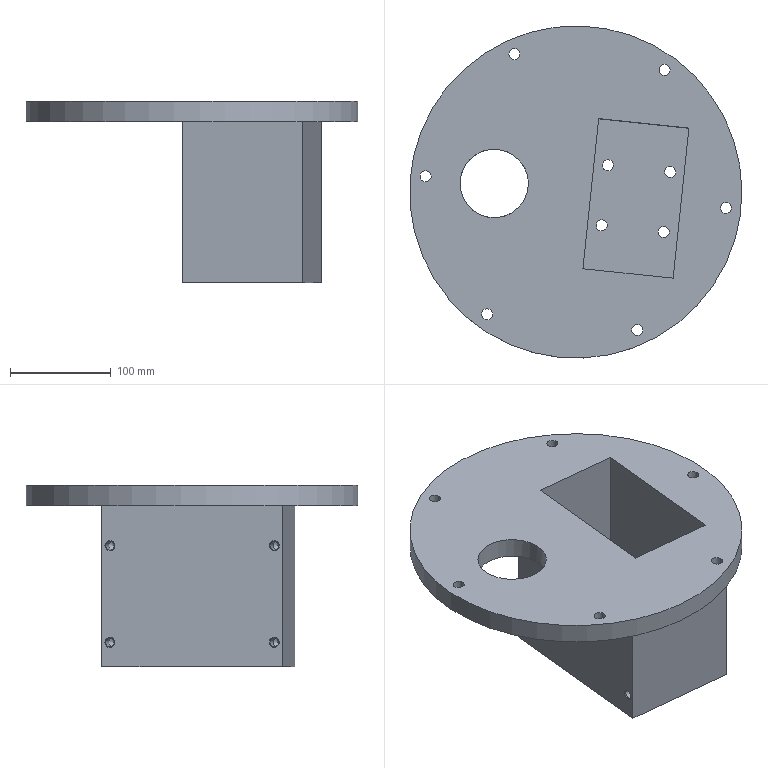Component | NX | CONN_SUPPORT | 1 solid | 36 faces | volume 2842323 mm3 | cylinder 16 | plane 12 | cone 8 | commonest cylinder face diameters 11 x10 8.5 x4 330 x1 68 x1